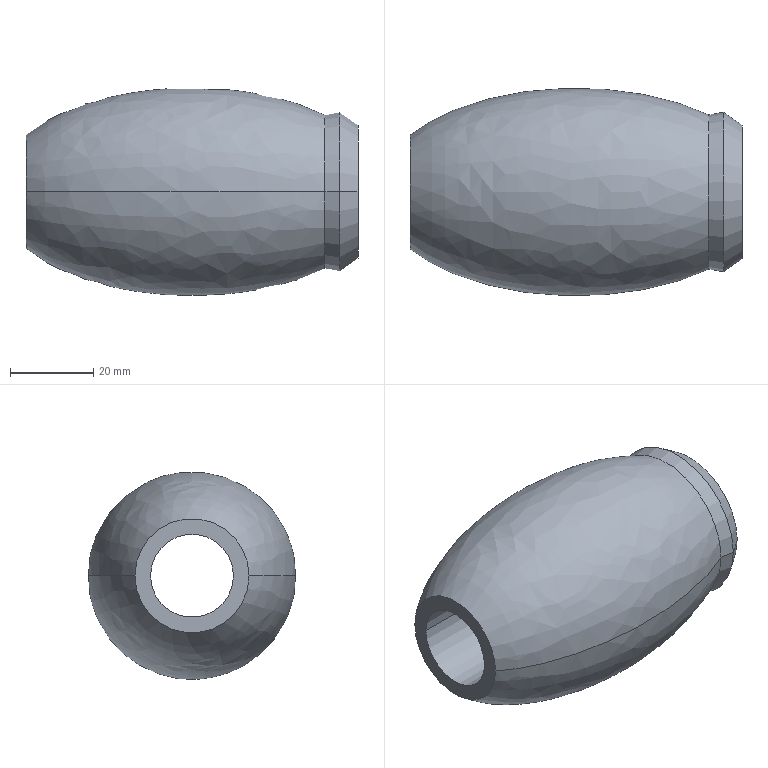Component | SolidWorks | 1-1 | 1 solid | 10 faces | box 80 x 50 x 50 mm | volume 97007 mm3 | cone 4 | spline 2 | cylinder 2 | plane 2 | commonest cylinder face diameters 20 x2
build123d program:
from build123d import *

# Parameters (mm, degrees)
SKETCH2_R           = 20
SKETCH2_R_2         = 13.758
BOSS_EXTRUDE2_DEPTH = 9.864
BOSS_EXTRUDE2_DRAFT = -10
CHAMFER2_SIZE       = 4.5
CHAMFER2_SIZE2      = 3.884


with BuildPart() as part:
    # Sketch1 → Revolve2 (revolve)
    with BuildSketch(Plane.XY, mode=Mode.PRIVATE) as revolve2_sk:
        with BuildLine():
            Line((-40, 10), (40, 10))
            add(Edge.make_bspline(
                [(40, 10), (0, 48.4), (-40, 10)],
                knots=[0.4719, 0.4719, 0.4719, 2.67, 2.67, 2.67], degree=2, weights=[1, 0.4545, 1]))
        make_face()
        with BuildLine():
            Line((-40, 13.758), (-40, 10))
            add(Edge.make_bspline(
                [(40, 10), (0, 48.4), (-40, 10)],
                knots=[0.4719, 0.4719, 0.4719, 2.67, 2.67, 2.67], degree=2, weights=[1, 0.4545, 1]))
            Line((40, 10), (40, 13.758))
            add(Edge.make_bspline(
                [(40, 13.758), (25.801, 25), (0, 25)],
                knots=[0.5828, 0.5828, 0.5828, 1.571, 1.571, 1.571], degree=2, weights=[1, 0.7752, 0.7752]))
            add(Edge.make_bspline(
                [(0, 25), (-25.801, 25), (-40, 13.758)],
                knots=[1.571, 1.571, 1.571, 2.559, 2.559, 2.559], degree=2, weights=[0.7752, 0.7752, 1]))
        make_face()
    revolve(revolve2_sk.sketch.rotate(Axis((42.753, 0, 0), (1, 0, 0)), 180), axis=Axis((42.753, 0, 0), (1, 0, 0)))


with BuildPart() as boss_extrude2_tool:
    # Sketch2 → Boss-Extrude2 (with draft: the straight prism first)
    with BuildSketch(Plane(origin=(40, 0, 0), x_dir=(0, 0, -1), z_dir=(1, 0, 0))):
        Circle(SKETCH2_R)
        Circle(SKETCH2_R_2, mode=Mode.SUBTRACT)
    extrude(amount=-BOSS_EXTRUDE2_DEPTH)
    # Boss-Extrude2: the draft: its side faces are tilted about the plane it starts from
    boss_extrude2_sides = [boss_extrude2_tool.faces().sort_by_distance(p)[0] for p in [
        (35.068, 0, 20),
        (35.068, 0, 13.758),
    ]]
    draft(boss_extrude2_sides, Plane(origin=(40, 0, 0), x_dir=(0, 0, -1), z_dir=(1, 0, 0)), BOSS_EXTRUDE2_DRAFT)


with BuildPart() as part_1:
    add(part.part)

    # Boss-Extrude2: add boss_extrude2_tool
    add(boss_extrude2_tool.part)

    # Chamfer2
    chamfer2_edges = [part_1.edges().sort_by_distance(p)[0] for p in [
        (40, 0, 20),
    ]]
    chamfer2_side = [part_1.faces().sort_by_distance(p)[0] for p in [
        (36.012, 0, 19.297),
    ]]
    chamfer(chamfer2_edges, length=CHAMFER2_SIZE, length2=CHAMFER2_SIZE2, reference=chamfer2_side[0])


solid = part_1.part

# Placed as in the assembly
solid = solid.moved(Location((-18.671, 8.534, 0), (0, 0, 0)))
STEP:
#1=COLOUR_RGB('',0.7922,0.8196,0.9333);
#2=FILL_AREA_STYLE_COLOUR('',#1);
#3=FILL_AREA_STYLE('',(#2));
#4=SURFACE_STYLE_FILL_AREA(#3);
#5=SURFACE_SIDE_STYLE('',(#4));
#6=SURFACE_STYLE_USAGE(.BOTH.,#5);
#7=PRESENTATION_STYLE_ASSIGNMENT((#6));
#8=CARTESIAN_POINT('',(0.5257,-0.3961,0.));
#9=VERTEX_POINT('',#8);
#10=CARTESIAN_POINT('',(0.5257,1.068,0.));
#11=VERTEX_POINT('',#10);
#12=CARTESIAN_POINT('',(0.5257,0.336,0.));
#13=DIRECTION('',(1.,-0.,0.));
#14=DIRECTION('',(-0.,-1.,0.));
#15=AXIS2_PLACEMENT_3D('',#12,#13,#14);
#16=CIRCLE('',#15,0.732);
#17=EDGE_CURVE('',#9,#11,#16,.T.);
#18=ORIENTED_EDGE('',*,*,#17,.F.);
#19=CARTESIAN_POINT('',(-2.31,-0.2057,-0.));
#20=VERTEX_POINT('',#19);
#21=CARTESIAN_POINT('',(0.5257,-0.3961,0.));
#22=CARTESIAN_POINT('',(-0.3969,-0.8288,-0.));
#23=CARTESIAN_POINT('',(-1.627,-0.7462,-0.));
#24=CARTESIAN_POINT('',(-2.31,-0.2057,-0.));
#25=(BOUNDED_CURVE()B_SPLINE_CURVE(3,(#21,#22,#23,#24),.UNSPECIFIED.,.F.,.F.)B_SPLINE_CURVE_WITH_KNOTS((4,4),(3.98,5.7),.UNSPECIFIED.)CURVE()GEOMETRIC_REPRESENTATION_ITEM()RATIONAL_B_SPLINE_CURVE((1.,0.7682,0.7682,1.))REPRESENTATION_ITEM(''));
#26=EDGE_CURVE('',#9,#20,#25,.T.);
#27=ORIENTED_EDGE('',*,*,#26,.T.);
#28=CARTESIAN_POINT('',(-2.31,0.8776,0.));
#29=VERTEX_POINT('',#28);
#30=CARTESIAN_POINT('',(-2.31,0.336,0.));
#31=DIRECTION('',(-1.,0.,0.));
#32=DIRECTION('',(0.,-1.,0.));
#33=AXIS2_PLACEMENT_3D('',#30,#31,#32);
#34=CIRCLE('',#33,0.5417);
#35=EDGE_CURVE('',#29,#20,#34,.T.);
#36=ORIENTED_EDGE('',*,*,#35,.F.);
#37=CARTESIAN_POINT('',(0.5257,1.068,0.));
#38=CARTESIAN_POINT('',(-0.3969,1.501,0.));
#39=CARTESIAN_POINT('',(-1.627,1.418,0.));
#40=CARTESIAN_POINT('',(-2.31,0.8776,0.));
#41=(BOUNDED_CURVE()B_SPLINE_CURVE(3,(#37,#38,#39,#40),.UNSPECIFIED.,.F.,.F.)B_SPLINE_CURVE_WITH_KNOTS((4,4),(3.98,5.7),.UNSPECIFIED.)CURVE()GEOMETRIC_REPRESENTATION_ITEM()RATIONAL_B_SPLINE_CURVE((1.,0.7682,0.7682,1.))REPRESENTATION_ITEM(''));
#42=EDGE_CURVE('',#11,#29,#41,.T.);
#43=ORIENTED_EDGE('',*,*,#42,.F.);
#44=EDGE_LOOP('',(#18,#27,#36,#43));
#45=FACE_OUTER_BOUND('',#44,.T.);
#46=CARTESIAN_POINT('',(0.5257,1.068,0.));
#47=CARTESIAN_POINT('',(0.5257,1.068,-1.464));
#48=CARTESIAN_POINT('',(0.5257,-0.3961,-1.464));
#49=CARTESIAN_POINT('',(0.5257,-0.3961,-0.));
#50=CARTESIAN_POINT('',(-0.3969,1.501,0.));
#51=CARTESIAN_POINT('',(-0.3969,1.501,-2.329));
#52=CARTESIAN_POINT('',(-0.3969,-0.8288,-2.329));
#53=CARTESIAN_POINT('',(-0.3969,-0.8288,-0.));
#54=CARTESIAN_POINT('',(-1.627,1.418,0.));
#55=CARTESIAN_POINT('',(-1.627,1.418,-2.164));
#56=CARTESIAN_POINT('',(-1.627,-0.7462,-2.164));
#57=CARTESIAN_POINT('',(-1.627,-0.7462,-0.));
#58=CARTESIAN_POINT('',(-2.31,0.8776,0.));
#59=CARTESIAN_POINT('',(-2.31,0.8776,-1.083));
#60=CARTESIAN_POINT('',(-2.31,-0.2057,-1.083));
#61=CARTESIAN_POINT('',(-2.31,-0.2057,-0.));
#62=(BOUNDED_SURFACE()B_SPLINE_SURFACE(3,3,((#46,#47,#48,#49),(#50,#51,#52,#53),(#54,#55,#56,#57),(#58,#59,#60,#61)),.UNSPECIFIED.,.F.,.F.,.T.)B_SPLINE_SURFACE_WITH_KNOTS((4,4),(4,4),(0.,1.),(0.,1.),.UNSPECIFIED.)GEOMETRIC_REPRESENTATION_ITEM()RATIONAL_B_SPLINE_SURFACE(((1.,0.3333,0.3333,1.),(0.7682,0.2561,0.2561,0.7682),(0.7682,0.2561,0.2561,0.7682),(1.,0.3333,0.3333,1.)))REPRESENTATION_ITEM('')SURFACE());
#63=ADVANCED_FACE('',(#45),#62,.F.);
#64=CARTESIAN_POINT('',(0.8397,0.9705,0.));
#65=VERTEX_POINT('',#64);
#66=CARTESIAN_POINT('',(0.8397,-0.2985,0.));
#67=VERTEX_POINT('',#66);
#68=CARTESIAN_POINT('',(0.8397,0.336,0.));
#69=DIRECTION('',(1.,-0.,0.));
#70=DIRECTION('',(0.,1.,0.));
#71=AXIS2_PLACEMENT_3D('',#68,#69,#70);
#72=CIRCLE('',#71,0.6345);
#73=EDGE_CURVE('',#65,#67,#72,.T.);
#74=ORIENTED_EDGE('',*,*,#73,.F.);
#75=CARTESIAN_POINT('',(0.6653,1.093,0.));
#76=VERTEX_POINT('',#75);
#77=CARTESIAN_POINT('',(0.8397,0.9705,0.));
#78=DIRECTION('',(-0.8192,0.5736,0.));
#79=VECTOR('',#78,39.37);
#80=LINE('',#77,#79);
#81=EDGE_CURVE('',#65,#76,#80,.T.);
#82=ORIENTED_EDGE('',*,*,#81,.T.);
#83=CARTESIAN_POINT('',(0.6653,-0.4207,0.));
#84=VERTEX_POINT('',#83);
#85=CARTESIAN_POINT('',(0.6653,0.336,0.));
#86=DIRECTION('',(-1.,0.,0.));
#87=DIRECTION('',(-0.,-1.,0.));
#88=AXIS2_PLACEMENT_3D('',#85,#86,#87);
#89=CIRCLE('',#88,0.7566);
#90=EDGE_CURVE('',#84,#76,#89,.T.);
#91=ORIENTED_EDGE('',*,*,#90,.F.);
#92=CARTESIAN_POINT('',(0.8397,-0.2985,0.));
#93=DIRECTION('',(-0.8192,-0.5736,0.));
#94=VECTOR('',#93,39.37);
#95=LINE('',#92,#94);
#96=EDGE_CURVE('',#67,#84,#95,.T.);
#97=ORIENTED_EDGE('',*,*,#96,.F.);
#98=EDGE_LOOP('',(#74,#82,#91,#97));
#99=FACE_OUTER_BOUND('',#98,.T.);
#100=CARTESIAN_POINT('',(0.8397,0.336,0.));
#101=DIRECTION('',(-1.,0.,0.));
#102=DIRECTION('',(-0.,-1.,0.));
#103=AXIS2_PLACEMENT_3D('',#100,#101,#102);
#104=CONICAL_SURFACE('',#103,0.6345,0.6109);
#105=ADVANCED_FACE('',(#99),#104,.T.);
#106=CARTESIAN_POINT('',(0.5257,0.336,0.));
#107=DIRECTION('',(1.,-0.,0.));
#108=DIRECTION('',(-0.,-1.,0.));
#109=AXIS2_PLACEMENT_3D('',#106,#107,#108);
#110=CIRCLE('',#109,0.732);
#111=EDGE_CURVE('',#11,#9,#110,.T.);
#112=ORIENTED_EDGE('',*,*,#111,.T.);
#113=CARTESIAN_POINT('',(0.8397,-0.4514,0.));
#114=DIRECTION('',(0.9848,-0.1736,0.));
#115=VECTOR('',#114,39.37);
#116=LINE('',#113,#115);
#117=EDGE_CURVE('',#9,#84,#116,.T.);
#118=ORIENTED_EDGE('',*,*,#117,.T.);
#119=ORIENTED_EDGE('',*,*,#90,.T.);
#120=CARTESIAN_POINT('',(0.8397,1.123,0.));
#121=DIRECTION('',(0.9848,0.1736,0.));
#122=VECTOR('',#121,39.37);
#123=LINE('',#120,#122);
#124=EDGE_CURVE('',#11,#76,#123,.T.);
#125=ORIENTED_EDGE('',*,*,#124,.F.);
#126=EDGE_LOOP('',(#112,#118,#119,#125));
#127=FACE_OUTER_BOUND('',#126,.T.);
#128=CARTESIAN_POINT('',(0.8397,0.336,0.));
#129=DIRECTION('',(1.,-0.,0.));
#130=DIRECTION('',(0.,1.,0.));
#131=AXIS2_PLACEMENT_3D('',#128,#129,#130);
#132=CONICAL_SURFACE('',#131,0.7874,0.1745);
#133=ADVANCED_FACE('',(#127),#132,.T.);
#134=CARTESIAN_POINT('',(0.8397,0.7297,0.));
#135=VERTEX_POINT('',#134);
#136=CARTESIAN_POINT('',(0.8397,-0.05772,0.));
#137=VERTEX_POINT('',#136);
#138=CARTESIAN_POINT('',(0.8397,0.336,0.));
#139=DIRECTION('',(-1.,0.,0.));
#140=DIRECTION('',(-0.,-1.,0.));
#141=AXIS2_PLACEMENT_3D('',#138,#139,#140);
#142=CIRCLE('',#141,0.3937);
#143=EDGE_CURVE('',#135,#137,#142,.T.);
#144=ORIENTED_EDGE('',*,*,#143,.F.);
#145=CARTESIAN_POINT('',(-2.31,0.7297,0.));
#146=VERTEX_POINT('',#145);
#147=CARTESIAN_POINT('',(0.9481,0.7297,0.));
#148=DIRECTION('',(-1.,0.,0.));
#149=VECTOR('',#148,39.37);
#150=LINE('',#147,#149);
#151=EDGE_CURVE('',#135,#146,#150,.T.);
#152=ORIENTED_EDGE('',*,*,#151,.T.);
#153=CARTESIAN_POINT('',(-2.31,-0.05772,0.));
#154=VERTEX_POINT('',#153);
#155=CARTESIAN_POINT('',(-2.31,0.336,0.));
#156=DIRECTION('',(-1.,0.,0.));
#157=DIRECTION('',(0.,-1.,0.));
#158=AXIS2_PLACEMENT_3D('',#155,#156,#157);
#159=CIRCLE('',#158,0.3937);
#160=EDGE_CURVE('',#146,#154,#159,.T.);
#161=ORIENTED_EDGE('',*,*,#160,.T.);
#162=CARTESIAN_POINT('',(0.9481,-0.05772,0.));
#163=DIRECTION('',(-1.,0.,0.));
#164=VECTOR('',#163,39.37);
#165=LINE('',#162,#164);
#166=EDGE_CURVE('',#137,#154,#165,.T.);
#167=ORIENTED_EDGE('',*,*,#166,.F.);
#168=EDGE_LOOP('',(#144,#152,#161,#167));
#169=FACE_OUTER_BOUND('',#168,.T.);
#170=CARTESIAN_POINT('',(0.9481,0.336,0.));
#171=DIRECTION('',(-1.,0.,0.));
#172=DIRECTION('',(-0.,-1.,0.));
#173=AXIS2_PLACEMENT_3D('',#170,#171,#172);
#174=CYLINDRICAL_SURFACE('',#173,0.3937);
#175=ADVANCED_FACE('',(#169),#174,.F.);
#176=ORIENTED_EDGE('',*,*,#151,.F.);
#177=CARTESIAN_POINT('',(0.8397,0.336,0.));
#178=DIRECTION('',(-1.,0.,0.));
#179=DIRECTION('',(-0.,-1.,0.));
#180=AXIS2_PLACEMENT_3D('',#177,#178,#179);
#181=CIRCLE('',#180,0.3937);
#182=EDGE_CURVE('',#137,#135,#181,.T.);
#183=ORIENTED_EDGE('',*,*,#182,.F.);
#184=ORIENTED_EDGE('',*,*,#166,.T.);
#185=CARTESIAN_POINT('',(-2.31,0.336,0.));
#186=DIRECTION('',(-1.,0.,0.));
#187=DIRECTION('',(0.,-1.,0.));
#188=AXIS2_PLACEMENT_3D('',#185,#186,#187);
#189=CIRCLE('',#188,0.3937);
#190=EDGE_CURVE('',#154,#146,#189,.T.);
#191=ORIENTED_EDGE('',*,*,#190,.T.);
#192=EDGE_LOOP('',(#176,#183,#184,#191));
#193=FACE_OUTER_BOUND('',#192,.T.);
#194=CARTESIAN_POINT('',(0.9481,0.336,0.));
#195=DIRECTION('',(-1.,0.,0.));
#196=DIRECTION('',(-0.,-1.,0.));
#197=AXIS2_PLACEMENT_3D('',#194,#195,#196);
#198=CYLINDRICAL_SURFACE('',#197,0.3937);
#199=ADVANCED_FACE('',(#193),#198,.F.);
#200=CARTESIAN_POINT('',(0.8397,0.336,0.));
#201=DIRECTION('',(1.,-0.,0.));
#202=DIRECTION('',(0.,1.,0.));
#203=AXIS2_PLACEMENT_3D('',#200,#201,#202);
#204=CIRCLE('',#203,0.6345);
#205=EDGE_CURVE('',#67,#65,#204,.T.);
#206=ORIENTED_EDGE('',*,*,#205,.T.);
#207=ORIENTED_EDGE('',*,*,#73,.T.);
#208=EDGE_LOOP('',(#206,#207));
#209=FACE_OUTER_BOUND('',#208,.T.);
#210=ORIENTED_EDGE('',*,*,#182,.T.);
#211=ORIENTED_EDGE('',*,*,#143,.T.);
#212=EDGE_LOOP('',(#210,#211));
#213=FACE_BOUND('',#212,.T.);
#214=CARTESIAN_POINT('',(0.8397,0.336,0.));
#215=DIRECTION('',(1.,-0.,0.));
#216=DIRECTION('',(0.,1.,0.));
#217=AXIS2_PLACEMENT_3D('',#214,#215,#216);
#218=PLANE('',#217);
#219=ADVANCED_FACE('',(#209,#213),#218,.T.);
#220=ORIENTED_EDGE('',*,*,#26,.F.);
#221=ORIENTED_EDGE('',*,*,#111,.F.);
#222=ORIENTED_EDGE('',*,*,#42,.T.);
#223=CARTESIAN_POINT('',(-2.31,0.336,0.));
#224=DIRECTION('',(-1.,0.,0.));
#225=DIRECTION('',(0.,-1.,0.));
#226=AXIS2_PLACEMENT_3D('',#223,#224,#225);
#227=CIRCLE('',#226,0.5417);
#228=EDGE_CURVE('',#20,#29,#227,.T.);
#229=ORIENTED_EDGE('',*,*,#228,.F.);
#230=EDGE_LOOP('',(#220,#221,#222,#229));
#231=FACE_OUTER_BOUND('',#230,.T.);
#232=CARTESIAN_POINT('',(0.5257,-0.3961,-0.));
#233=CARTESIAN_POINT('',(0.5257,-0.3961,1.464));
#234=CARTESIAN_POINT('',(0.5257,1.068,1.464));
#235=CARTESIAN_POINT('',(0.5257,1.068,0.));
#236=CARTESIAN_POINT('',(-0.3969,-0.8288,-0.));
#237=CARTESIAN_POINT('',(-0.3969,-0.8288,2.329));
#238=CARTESIAN_POINT('',(-0.3969,1.501,2.329));
#239=CARTESIAN_POINT('',(-0.3969,1.501,0.));
#240=CARTESIAN_POINT('',(-1.627,-0.7462,-0.));
#241=CARTESIAN_POINT('',(-1.627,-0.7462,2.164));
#242=CARTESIAN_POINT('',(-1.627,1.418,2.164));
#243=CARTESIAN_POINT('',(-1.627,1.418,0.));
#244=CARTESIAN_POINT('',(-2.31,-0.2057,-0.));
#245=CARTESIAN_POINT('',(-2.31,-0.2057,1.083));
#246=CARTESIAN_POINT('',(-2.31,0.8776,1.083));
#247=CARTESIAN_POINT('',(-2.31,0.8776,0.));
#248=(BOUNDED_SURFACE()B_SPLINE_SURFACE(3,3,((#232,#233,#234,#235),(#236,#237,#238,#239),(#240,#241,#242,#243),(#244,#245,#246,#247)),.UNSPECIFIED.,.F.,.F.,.F.)B_SPLINE_SURFACE_WITH_KNOTS((4,4),(4,4),(0.,1.),(0.,1.),.UNSPECIFIED.)GEOMETRIC_REPRESENTATION_ITEM()RATIONAL_B_SPLINE_SURFACE(((1.,0.3333,0.3333,1.),(0.7682,0.2561,0.2561,0.7682),(0.7682,0.2561,0.2561,0.7682),(1.,0.3333,0.3333,1.)))REPRESENTATION_ITEM('')SURFACE());
#249=ADVANCED_FACE('',(#231),#248,.F.);
#250=ORIENTED_EDGE('',*,*,#190,.F.);
#251=ORIENTED_EDGE('',*,*,#160,.F.);
#252=EDGE_LOOP('',(#250,#251));
#253=FACE_BOUND('',#252,.T.);
#254=ORIENTED_EDGE('',*,*,#35,.T.);
#255=ORIENTED_EDGE('',*,*,#228,.T.);
#256=EDGE_LOOP('',(#254,#255));
#257=FACE_OUTER_BOUND('',#256,.T.);
#258=CARTESIAN_POINT('',(-2.31,0.336,0.));
#259=DIRECTION('',(1.,-0.,0.));
#260=DIRECTION('',(0.,1.,0.));
#261=AXIS2_PLACEMENT_3D('',#258,#259,#260);
#262=PLANE('',#261);
#263=ADVANCED_FACE('',(#253,#257),#262,.F.);
#264=ORIENTED_EDGE('',*,*,#117,.F.);
#265=ORIENTED_EDGE('',*,*,#17,.T.);
#266=ORIENTED_EDGE('',*,*,#124,.T.);
#267=CARTESIAN_POINT('',(0.6653,0.336,0.));
#268=DIRECTION('',(-1.,0.,0.));
#269=DIRECTION('',(-0.,-1.,0.));
#270=AXIS2_PLACEMENT_3D('',#267,#268,#269);
#271=CIRCLE('',#270,0.7566);
#272=EDGE_CURVE('',#76,#84,#271,.T.);
#273=ORIENTED_EDGE('',*,*,#272,.T.);
#274=EDGE_LOOP('',(#264,#265,#266,#273));
#275=FACE_OUTER_BOUND('',#274,.T.);
#276=CARTESIAN_POINT('',(0.8397,0.336,0.));
#277=DIRECTION('',(1.,-0.,0.));
#278=DIRECTION('',(0.,1.,0.));
#279=AXIS2_PLACEMENT_3D('',#276,#277,#278);
#280=CONICAL_SURFACE('',#279,0.7874,0.1745);
#281=ADVANCED_FACE('',(#275),#280,.T.);
#282=ORIENTED_EDGE('',*,*,#81,.F.);
#283=ORIENTED_EDGE('',*,*,#205,.F.);
#284=ORIENTED_EDGE('',*,*,#96,.T.);
#285=ORIENTED_EDGE('',*,*,#272,.F.);
#286=EDGE_LOOP('',(#282,#283,#284,#285));
#287=FACE_OUTER_BOUND('',#286,.T.);
#288=CARTESIAN_POINT('',(0.8397,0.336,0.));
#289=DIRECTION('',(-1.,0.,0.));
#290=DIRECTION('',(-0.,-1.,0.));
#291=AXIS2_PLACEMENT_3D('',#288,#289,#290);
#292=CONICAL_SURFACE('',#291,0.6345,0.6109);
#293=ADVANCED_FACE('',(#287),#292,.T.);
#294=CLOSED_SHELL('',(#63,#105,#133,#175,#199,#219,#249,#263,#281,#293));
#295=MANIFOLD_SOLID_BREP('',#294);
#296=STYLED_ITEM('',(#7),#295);
#297=(LENGTH_UNIT()NAMED_UNIT(*)SI_UNIT($,.METRE.));
#298=LENGTH_MEASURE_WITH_UNIT(LENGTH_MEASURE(0.0254),#297);
#299=DIMENSIONAL_EXPONENTS(1.,0.,0.,0.,0.,0.,0.);
#300=(CONVERSION_BASED_UNIT('',#298)LENGTH_UNIT()NAMED_UNIT(#299));
#301=UNCERTAINTY_MEASURE_WITH_UNIT(LENGTH_MEASURE(0.00001),#300,'','');
#302=(NAMED_UNIT(*)PLANE_ANGLE_UNIT()SI_UNIT($,.RADIAN.));
#303=(NAMED_UNIT(*)SI_UNIT($,.STERADIAN.)SOLID_ANGLE_UNIT());
#304=(GEOMETRIC_REPRESENTATION_CONTEXT(3)GLOBAL_UNCERTAINTY_ASSIGNED_CONTEXT((#301))GLOBAL_UNIT_ASSIGNED_CONTEXT((#300,#302,#303))REPRESENTATION_CONTEXT('',''));
#305=MECHANICAL_DESIGN_GEOMETRIC_PRESENTATION_REPRESENTATION('',(#296),#304);
#306=CARTESIAN_POINT('',(0.,0.,0.));
#307=DIRECTION('',(0.,0.,1.));
#308=DIRECTION('',(1.,0.,0.));
#309=AXIS2_PLACEMENT_3D('',#306,#307,#308);
#310=(LENGTH_UNIT()NAMED_UNIT(*)SI_UNIT($,.METRE.));
#311=LENGTH_MEASURE_WITH_UNIT(LENGTH_MEASURE(0.0254),#310);
#312=DIMENSIONAL_EXPONENTS(1.,0.,0.,0.,0.,0.,0.);
#313=(CONVERSION_BASED_UNIT('',#311)LENGTH_UNIT()NAMED_UNIT(#312));
#314=UNCERTAINTY_MEASURE_WITH_UNIT(LENGTH_MEASURE(0.00001),#313,'','');
#315=(NAMED_UNIT(*)PLANE_ANGLE_UNIT()SI_UNIT($,.RADIAN.));
#316=(NAMED_UNIT(*)SI_UNIT($,.STERADIAN.)SOLID_ANGLE_UNIT());
#317=(GEOMETRIC_REPRESENTATION_CONTEXT(3)GLOBAL_UNCERTAINTY_ASSIGNED_CONTEXT((#314))GLOBAL_UNIT_ASSIGNED_CONTEXT((#313,#315,#316))REPRESENTATION_CONTEXT('',''));
#318=ADVANCED_BREP_SHAPE_REPRESENTATION('',(#295,#309),#317);
#319=PRESENTATION_LAYER_ASSIGNMENT('','',(#296));